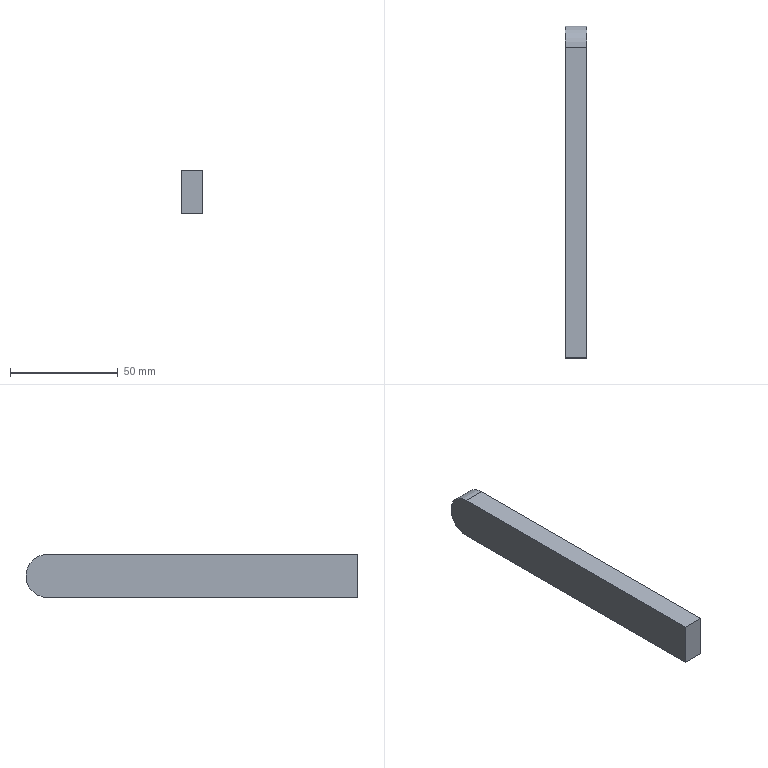Component | SolidWorks | LimitRod-1 | 1 solid | 7 faces | box 10 x 154 x 20 mm | volume 30371 mm3 | plane 5 | cylinder 2 | commonest cylinder face diameters 20 x2
build123d program:
from build123d import *

# Parameters (mm, degrees)
BOSS_EXTRUDE1_DEPTH = 10


with BuildPart() as part:
    # Sketch2 → Boss-Extrude1 (new body)
    with BuildSketch(Plane.XY):
        with BuildLine():
            Line((-299.131, 69.185), (-156.628, 48.48))
            ThreePointArc((-156.628, 48.48), (-148.169, 37.146), (-159.503, 28.687))
            Line((-159.503, 28.687), (-302.007, 49.393))
            Line((-302.007, 49.393), (-299.131, 69.185))
        make_face()
    extrude(amount=-BOSS_EXTRUDE1_DEPTH)


solid = part.part

# Placed as in the assembly
solid = solid.moved(Location((-513.446, 158.319, 305.916), (98.267, 90, 0)))
STEP:
#1=COLOUR_RGB('',0.7922,0.8196,0.9333);
#2=FILL_AREA_STYLE_COLOUR('',#1);
#3=FILL_AREA_STYLE('',(#2));
#4=SURFACE_STYLE_FILL_AREA(#3);
#5=SURFACE_SIDE_STYLE('',(#4));
#6=SURFACE_STYLE_USAGE(.BOTH.,#5);
#7=PRESENTATION_STYLE_ASSIGNMENT((#6));
#8=CARTESIAN_POINT('',(-20.608,-0.1438,12.259));
#9=VERTEX_POINT('',#8);
#10=CARTESIAN_POINT('',(-20.608,0.2459,12.709));
#11=VERTEX_POINT('',#10);
#12=CARTESIAN_POINT('',(-20.608,-0.1438,12.652));
#13=DIRECTION('',(1.,-0.,0.));
#14=DIRECTION('',(0.,-0.9896,-0.1438));
#15=AXIS2_PLACEMENT_3D('',#12,#13,#14);
#16=CIRCLE('',#15,0.3937);
#17=EDGE_CURVE('',#9,#11,#16,.T.);
#18=ORIENTED_EDGE('',*,*,#17,.T.);
#19=CARTESIAN_POINT('',(-20.214,0.2459,12.709));
#20=VERTEX_POINT('',#19);
#21=CARTESIAN_POINT('',(-20.608,0.2459,12.709));
#22=DIRECTION('',(1.,-0.,0.));
#23=VECTOR('',#22,39.37);
#24=LINE('',#21,#23);
#25=EDGE_CURVE('',#11,#20,#24,.T.);
#26=ORIENTED_EDGE('',*,*,#25,.T.);
#27=CARTESIAN_POINT('',(-20.214,-0.1438,12.259));
#28=VERTEX_POINT('',#27);
#29=CARTESIAN_POINT('',(-20.214,-0.1438,12.652));
#30=DIRECTION('',(1.,-0.,0.));
#31=DIRECTION('',(0.,-0.9896,-0.1438));
#32=AXIS2_PLACEMENT_3D('',#29,#30,#31);
#33=CIRCLE('',#32,0.3937);
#34=EDGE_CURVE('',#28,#20,#33,.T.);
#35=ORIENTED_EDGE('',*,*,#34,.F.);
#36=CARTESIAN_POINT('',(-20.608,-0.1438,12.259));
#37=DIRECTION('',(1.,-0.,0.));
#38=VECTOR('',#37,39.37);
#39=LINE('',#36,#38);
#40=EDGE_CURVE('',#9,#28,#39,.T.);
#41=ORIENTED_EDGE('',*,*,#40,.F.);
#42=EDGE_LOOP('',(#18,#26,#35,#41));
#43=FACE_OUTER_BOUND('',#42,.T.);
#44=CARTESIAN_POINT('',(-20.608,-0.1438,12.652));
#45=DIRECTION('',(1.,-0.,0.));
#46=DIRECTION('',(0.,0.9896,0.1438));
#47=AXIS2_PLACEMENT_3D('',#44,#45,#46);
#48=CYLINDRICAL_SURFACE('',#47,0.3937);
#49=ADVANCED_FACE('',(#43),#48,.T.);
#50=CARTESIAN_POINT('',(-20.214,-5.813,13.046));
#51=VERTEX_POINT('',#50);
#52=CARTESIAN_POINT('',(-20.214,-5.813,12.259));
#53=VERTEX_POINT('',#52);
#54=CARTESIAN_POINT('',(-20.214,-5.813,13.046));
#55=DIRECTION('',(0.,-0.,-1.));
#56=VECTOR('',#55,39.37);
#57=LINE('',#54,#56);
#58=EDGE_CURVE('',#51,#53,#57,.T.);
#59=ORIENTED_EDGE('',*,*,#58,.F.);
#60=CARTESIAN_POINT('',(-20.608,-5.813,13.046));
#61=VERTEX_POINT('',#60);
#62=CARTESIAN_POINT('',(-20.608,-5.813,13.046));
#63=DIRECTION('',(1.,-0.,0.));
#64=VECTOR('',#63,39.37);
#65=LINE('',#62,#64);
#66=EDGE_CURVE('',#61,#51,#65,.T.);
#67=ORIENTED_EDGE('',*,*,#66,.F.);
#68=CARTESIAN_POINT('',(-20.608,-5.813,12.259));
#69=VERTEX_POINT('',#68);
#70=CARTESIAN_POINT('',(-20.608,-5.813,13.046));
#71=DIRECTION('',(0.,-0.,-1.));
#72=VECTOR('',#71,39.37);
#73=LINE('',#70,#72);
#74=EDGE_CURVE('',#61,#69,#73,.T.);
#75=ORIENTED_EDGE('',*,*,#74,.T.);
#76=CARTESIAN_POINT('',(-20.608,-5.813,12.259));
#77=DIRECTION('',(1.,-0.,0.));
#78=VECTOR('',#77,39.37);
#79=LINE('',#76,#78);
#80=EDGE_CURVE('',#69,#53,#79,.T.);
#81=ORIENTED_EDGE('',*,*,#80,.T.);
#82=EDGE_LOOP('',(#59,#67,#75,#81));
#83=FACE_OUTER_BOUND('',#82,.T.);
#84=CARTESIAN_POINT('',(-20.608,-5.813,13.046));
#85=DIRECTION('',(-0.,-1.,0.));
#86=DIRECTION('',(0.,-0.,-1.));
#87=AXIS2_PLACEMENT_3D('',#84,#85,#86);
#88=PLANE('',#87);
#89=ADVANCED_FACE('',(#83),#88,.T.);
#90=CARTESIAN_POINT('',(-20.214,-0.1438,13.046));
#91=VERTEX_POINT('',#90);
#92=CARTESIAN_POINT('',(-20.214,-5.813,13.046));
#93=DIRECTION('',(-0.,-1.,-0.));
#94=VECTOR('',#93,39.37);
#95=LINE('',#92,#94);
#96=EDGE_CURVE('',#91,#51,#95,.T.);
#97=ORIENTED_EDGE('',*,*,#96,.F.);
#98=CARTESIAN_POINT('',(-20.608,-0.1438,13.046));
#99=VERTEX_POINT('',#98);
#100=CARTESIAN_POINT('',(-20.608,-0.1438,13.046));
#101=DIRECTION('',(1.,-0.,0.));
#102=VECTOR('',#101,39.37);
#103=LINE('',#100,#102);
#104=EDGE_CURVE('',#99,#91,#103,.T.);
#105=ORIENTED_EDGE('',*,*,#104,.F.);
#106=CARTESIAN_POINT('',(-20.608,-5.813,13.046));
#107=DIRECTION('',(-0.,-1.,-0.));
#108=VECTOR('',#107,39.37);
#109=LINE('',#106,#108);
#110=EDGE_CURVE('',#99,#61,#109,.T.);
#111=ORIENTED_EDGE('',*,*,#110,.T.);
#112=ORIENTED_EDGE('',*,*,#66,.T.);
#113=EDGE_LOOP('',(#97,#105,#111,#112));
#114=FACE_OUTER_BOUND('',#113,.T.);
#115=CARTESIAN_POINT('',(-20.608,-5.813,13.046));
#116=DIRECTION('',(-0.,-0.,1.));
#117=DIRECTION('',(-0.,-1.,-0.));
#118=AXIS2_PLACEMENT_3D('',#115,#116,#117);
#119=PLANE('',#118);
#120=ADVANCED_FACE('',(#114),#119,.T.);
#121=ORIENTED_EDGE('',*,*,#25,.F.);
#122=CARTESIAN_POINT('',(-20.608,-0.1438,12.652));
#123=DIRECTION('',(1.,-0.,0.));
#124=DIRECTION('',(0.,-0.9896,-0.1438));
#125=AXIS2_PLACEMENT_3D('',#122,#123,#124);
#126=CIRCLE('',#125,0.3937);
#127=EDGE_CURVE('',#11,#99,#126,.T.);
#128=ORIENTED_EDGE('',*,*,#127,.T.);
#129=ORIENTED_EDGE('',*,*,#104,.T.);
#130=CARTESIAN_POINT('',(-20.214,-0.1438,12.652));
#131=DIRECTION('',(1.,-0.,0.));
#132=DIRECTION('',(0.,-0.9896,-0.1438));
#133=AXIS2_PLACEMENT_3D('',#130,#131,#132);
#134=CIRCLE('',#133,0.3937);
#135=EDGE_CURVE('',#20,#91,#134,.T.);
#136=ORIENTED_EDGE('',*,*,#135,.F.);
#137=EDGE_LOOP('',(#121,#128,#129,#136));
#138=FACE_OUTER_BOUND('',#137,.T.);
#139=CARTESIAN_POINT('',(-20.608,-0.1438,12.652));
#140=DIRECTION('',(1.,-0.,0.));
#141=DIRECTION('',(0.,0.9896,0.1438));
#142=AXIS2_PLACEMENT_3D('',#139,#140,#141);
#143=CYLINDRICAL_SURFACE('',#142,0.3937);
#144=ADVANCED_FACE('',(#138),#143,.T.);
#145=CARTESIAN_POINT('',(-20.214,-0.1438,12.259));
#146=DIRECTION('',(0.,1.,0.));
#147=VECTOR('',#146,39.37);
#148=LINE('',#145,#147);
#149=EDGE_CURVE('',#53,#28,#148,.T.);
#150=ORIENTED_EDGE('',*,*,#149,.F.);
#151=ORIENTED_EDGE('',*,*,#80,.F.);
#152=CARTESIAN_POINT('',(-20.608,-0.1438,12.259));
#153=DIRECTION('',(0.,1.,0.));
#154=VECTOR('',#153,39.37);
#155=LINE('',#152,#154);
#156=EDGE_CURVE('',#69,#9,#155,.T.);
#157=ORIENTED_EDGE('',*,*,#156,.T.);
#158=ORIENTED_EDGE('',*,*,#40,.T.);
#159=EDGE_LOOP('',(#150,#151,#157,#158));
#160=FACE_OUTER_BOUND('',#159,.T.);
#161=CARTESIAN_POINT('',(-20.608,-0.1438,12.259));
#162=DIRECTION('',(0.,0.,-1.));
#163=DIRECTION('',(0.,1.,0.));
#164=AXIS2_PLACEMENT_3D('',#161,#162,#163);
#165=PLANE('',#164);
#166=ADVANCED_FACE('',(#160),#165,.T.);
#167=ORIENTED_EDGE('',*,*,#74,.F.);
#168=ORIENTED_EDGE('',*,*,#110,.F.);
#169=ORIENTED_EDGE('',*,*,#127,.F.);
#170=ORIENTED_EDGE('',*,*,#17,.F.);
#171=ORIENTED_EDGE('',*,*,#156,.F.);
#172=EDGE_LOOP('',(#167,#168,#169,#170,#171));
#173=FACE_OUTER_BOUND('',#172,.T.);
#174=CARTESIAN_POINT('',(-20.608,-0.1438,12.652));
#175=DIRECTION('',(-1.,0.,-0.));
#176=DIRECTION('',(-0.,-0.9896,-0.1438));
#177=AXIS2_PLACEMENT_3D('',#174,#175,#176);
#178=PLANE('',#177);
#179=ADVANCED_FACE('',(#173),#178,.T.);
#180=ORIENTED_EDGE('',*,*,#58,.T.);
#181=ORIENTED_EDGE('',*,*,#149,.T.);
#182=ORIENTED_EDGE('',*,*,#34,.T.);
#183=ORIENTED_EDGE('',*,*,#135,.T.);
#184=ORIENTED_EDGE('',*,*,#96,.T.);
#185=EDGE_LOOP('',(#180,#181,#182,#183,#184));
#186=FACE_OUTER_BOUND('',#185,.T.);
#187=CARTESIAN_POINT('',(-20.214,-0.1438,12.652));
#188=DIRECTION('',(-1.,0.,-0.));
#189=DIRECTION('',(-0.,-0.9896,-0.1438));
#190=AXIS2_PLACEMENT_3D('',#187,#188,#189);
#191=PLANE('',#190);
#192=ADVANCED_FACE('',(#186),#191,.F.);
#193=CLOSED_SHELL('',(#49,#89,#120,#144,#166,#179,#192));
#194=MANIFOLD_SOLID_BREP('',#193);
#195=STYLED_ITEM('',(#7),#194);
#196=PRESENTATION_LAYER_ASSIGNMENT('','',(#195));
#197=(LENGTH_UNIT()NAMED_UNIT(*)SI_UNIT($,.METRE.));
#198=LENGTH_MEASURE_WITH_UNIT(LENGTH_MEASURE(0.0254),#197);
#199=DIMENSIONAL_EXPONENTS(1.,0.,0.,0.,0.,0.,0.);
#200=(CONVERSION_BASED_UNIT('',#198)LENGTH_UNIT()NAMED_UNIT(#199));
#201=UNCERTAINTY_MEASURE_WITH_UNIT(LENGTH_MEASURE(0.00001),#200,'','');
#202=(NAMED_UNIT(*)PLANE_ANGLE_UNIT()SI_UNIT($,.RADIAN.));
#203=(NAMED_UNIT(*)SI_UNIT($,.STERADIAN.)SOLID_ANGLE_UNIT());
#204=(GEOMETRIC_REPRESENTATION_CONTEXT(3)GLOBAL_UNCERTAINTY_ASSIGNED_CONTEXT((#201))GLOBAL_UNIT_ASSIGNED_CONTEXT((#200,#202,#203))REPRESENTATION_CONTEXT('',''));
#205=MECHANICAL_DESIGN_GEOMETRIC_PRESENTATION_REPRESENTATION('',(#195),#204);
#206=CARTESIAN_POINT('',(0.,0.,0.));
#207=DIRECTION('',(0.,0.,1.));
#208=DIRECTION('',(1.,0.,0.));
#209=AXIS2_PLACEMENT_3D('',#206,#207,#208);
#210=(LENGTH_UNIT()NAMED_UNIT(*)SI_UNIT($,.METRE.));
#211=LENGTH_MEASURE_WITH_UNIT(LENGTH_MEASURE(0.0254),#210);
#212=DIMENSIONAL_EXPONENTS(1.,0.,0.,0.,0.,0.,0.);
#213=(CONVERSION_BASED_UNIT('',#211)LENGTH_UNIT()NAMED_UNIT(#212));
#214=UNCERTAINTY_MEASURE_WITH_UNIT(LENGTH_MEASURE(0.00001),#213,'','');
#215=(NAMED_UNIT(*)PLANE_ANGLE_UNIT()SI_UNIT($,.RADIAN.));
#216=(NAMED_UNIT(*)SI_UNIT($,.STERADIAN.)SOLID_ANGLE_UNIT());
#217=(GEOMETRIC_REPRESENTATION_CONTEXT(3)GLOBAL_UNCERTAINTY_ASSIGNED_CONTEXT((#214))GLOBAL_UNIT_ASSIGNED_CONTEXT((#213,#215,#216))REPRESENTATION_CONTEXT('',''));
#218=ADVANCED_BREP_SHAPE_REPRESENTATION('',(#194,#209),#217);